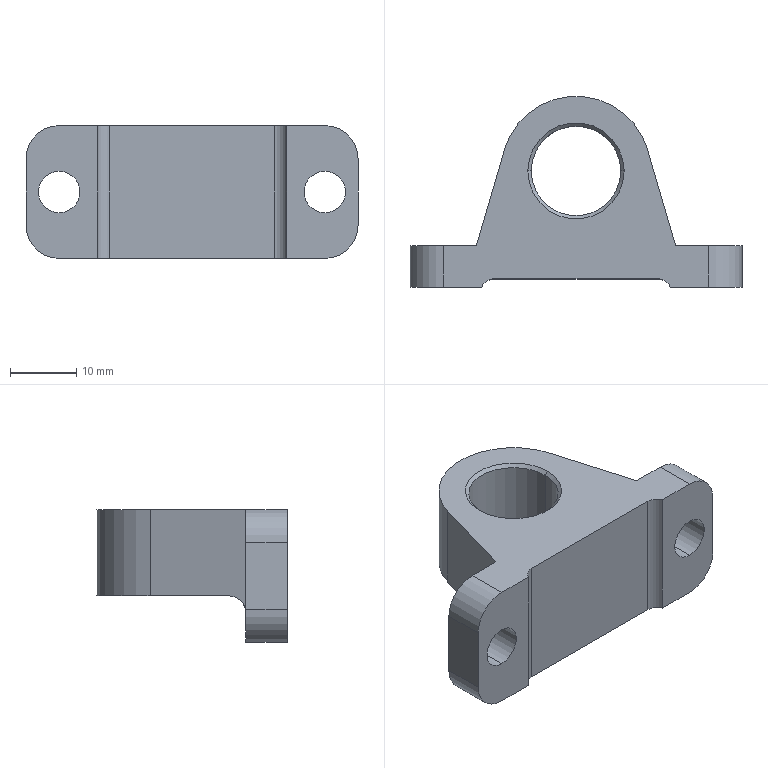Component | SolidWorks | CrankshaftSeat-1 | 1 solid | 29 faces | box 50 x 28.75 x 20 mm | volume 9719 mm3 | cylinder 14 | plane 11 | cone 4 | commonest cylinder face diameters 6.25 x4 10 x4 13.5 x2 4 x2 22.5 x1 5 x1
STEP:
#1=COLOUR_RGB('',0.7922,0.8196,0.9333);
#2=FILL_AREA_STYLE_COLOUR('',#1);
#3=FILL_AREA_STYLE('',(#2));
#4=SURFACE_STYLE_FILL_AREA(#3);
#5=SURFACE_SIDE_STYLE('',(#4));
#6=SURFACE_STYLE_USAGE(.BOTH.,#5);
#7=PRESENTATION_STYLE_ASSIGNMENT((#6));
#8=CARTESIAN_POINT('',(2.593,-9.906,9.939));
#9=VERTEX_POINT('',#8);
#10=CARTESIAN_POINT('',(3.125,-9.906,9.939));
#11=VERTEX_POINT('',#10);
#12=CARTESIAN_POINT('',(2.859,-9.906,9.939));
#13=DIRECTION('',(0.,0.,1.));
#14=DIRECTION('',(-1.,0.,0.));
#15=AXIS2_PLACEMENT_3D('',#12,#13,#14);
#16=CIRCLE('',#15,0.2657);
#17=EDGE_CURVE('',#9,#11,#16,.T.);
#18=ORIENTED_EDGE('',*,*,#17,.F.);
#19=CARTESIAN_POINT('',(2.573,-9.906,9.959));
#20=VERTEX_POINT('',#19);
#21=CARTESIAN_POINT('',(2.573,-9.906,9.959));
#22=DIRECTION('',(-0.7071,0.,0.7071));
#23=VECTOR('',#22,39.37);
#24=LINE('',#21,#23);
#25=EDGE_CURVE('',#9,#20,#24,.T.);
#26=ORIENTED_EDGE('',*,*,#25,.T.);
#27=CARTESIAN_POINT('',(3.144,-9.906,9.959));
#28=VERTEX_POINT('',#27);
#29=CARTESIAN_POINT('',(2.859,-9.906,9.959));
#30=DIRECTION('',(0.,0.,-1.));
#31=DIRECTION('',(-1.,0.,0.));
#32=AXIS2_PLACEMENT_3D('',#29,#30,#31);
#33=CIRCLE('',#32,0.2854);
#34=EDGE_CURVE('',#28,#20,#33,.T.);
#35=ORIENTED_EDGE('',*,*,#34,.F.);
#36=CARTESIAN_POINT('',(3.144,-9.906,9.959));
#37=DIRECTION('',(0.7071,0.,0.7071));
#38=VECTOR('',#37,39.37);
#39=LINE('',#36,#38);
#40=EDGE_CURVE('',#11,#28,#39,.T.);
#41=ORIENTED_EDGE('',*,*,#40,.F.);
#42=EDGE_LOOP('',(#18,#26,#35,#41));
#43=FACE_OUTER_BOUND('',#42,.T.);
#44=CARTESIAN_POINT('',(2.859,-9.906,9.959));
#45=DIRECTION('',(0.,0.,1.));
#46=DIRECTION('',(1.,0.,0.));
#47=AXIS2_PLACEMENT_3D('',#44,#45,#46);
#48=CONICAL_SURFACE('',#47,0.2854,0.7854);
#49=ADVANCED_FACE('',(#43),#48,.F.);
#50=CARTESIAN_POINT('',(3.125,-9.906,9.467));
#51=VERTEX_POINT('',#50);
#52=CARTESIAN_POINT('',(2.593,-9.906,9.467));
#53=VERTEX_POINT('',#52);
#54=CARTESIAN_POINT('',(2.859,-9.906,9.467));
#55=DIRECTION('',(0.,0.,-1.));
#56=DIRECTION('',(1.,0.,0.));
#57=AXIS2_PLACEMENT_3D('',#54,#55,#56);
#58=CIRCLE('',#57,0.2657);
#59=EDGE_CURVE('',#51,#53,#58,.T.);
#60=ORIENTED_EDGE('',*,*,#59,.F.);
#61=CARTESIAN_POINT('',(3.144,-9.906,9.447));
#62=VERTEX_POINT('',#61);
#63=CARTESIAN_POINT('',(3.144,-9.906,9.447));
#64=DIRECTION('',(0.7071,0.,-0.7071));
#65=VECTOR('',#64,39.37);
#66=LINE('',#63,#65);
#67=EDGE_CURVE('',#51,#62,#66,.T.);
#68=ORIENTED_EDGE('',*,*,#67,.T.);
#69=CARTESIAN_POINT('',(2.573,-9.906,9.447));
#70=VERTEX_POINT('',#69);
#71=CARTESIAN_POINT('',(2.859,-9.906,9.447));
#72=DIRECTION('',(0.,0.,1.));
#73=DIRECTION('',(1.,0.,0.));
#74=AXIS2_PLACEMENT_3D('',#71,#72,#73);
#75=CIRCLE('',#74,0.2854);
#76=EDGE_CURVE('',#70,#62,#75,.T.);
#77=ORIENTED_EDGE('',*,*,#76,.F.);
#78=CARTESIAN_POINT('',(2.573,-9.906,9.447));
#79=DIRECTION('',(-0.7071,0.,-0.7071));
#80=VECTOR('',#79,39.37);
#81=LINE('',#78,#80);
#82=EDGE_CURVE('',#53,#70,#81,.T.);
#83=ORIENTED_EDGE('',*,*,#82,.F.);
#84=EDGE_LOOP('',(#60,#68,#77,#83));
#85=FACE_OUTER_BOUND('',#84,.T.);
#86=CARTESIAN_POINT('',(2.859,-9.906,9.447));
#87=DIRECTION('',(0.,0.,-1.));
#88=DIRECTION('',(-1.,0.,0.));
#89=AXIS2_PLACEMENT_3D('',#86,#87,#88);
#90=CONICAL_SURFACE('',#89,0.2854,0.7854);
#91=ADVANCED_FACE('',(#85),#90,.F.);
#92=ORIENTED_EDGE('',*,*,#59,.T.);
#93=CARTESIAN_POINT('',(2.593,-9.906,9.447));
#94=DIRECTION('',(0.,0.,1.));
#95=VECTOR('',#94,39.37);
#96=LINE('',#93,#95);
#97=EDGE_CURVE('',#53,#9,#96,.T.);
#98=ORIENTED_EDGE('',*,*,#97,.T.);
#99=ORIENTED_EDGE('',*,*,#17,.T.);
#100=CARTESIAN_POINT('',(3.125,-9.906,9.447));
#101=DIRECTION('',(0.,0.,1.));
#102=VECTOR('',#101,39.37);
#103=LINE('',#100,#102);
#104=EDGE_CURVE('',#51,#11,#103,.T.);
#105=ORIENTED_EDGE('',*,*,#104,.F.);
#106=EDGE_LOOP('',(#92,#98,#99,#105));
#107=FACE_OUTER_BOUND('',#106,.T.);
#108=CARTESIAN_POINT('',(2.859,-9.906,9.447));
#109=DIRECTION('',(0.,0.,1.));
#110=DIRECTION('',(1.,0.,0.));
#111=AXIS2_PLACEMENT_3D('',#108,#109,#110);
#112=CYLINDRICAL_SURFACE('',#111,0.2657);
#113=ADVANCED_FACE('',(#107),#112,.F.);
#114=CARTESIAN_POINT('',(3.646,-10.594,9.442));
#115=VERTEX_POINT('',#114);
#116=CARTESIAN_POINT('',(3.646,-10.594,9.688));
#117=VERTEX_POINT('',#116);
#118=CARTESIAN_POINT('',(3.646,-10.594,9.565));
#119=DIRECTION('',(0.,1.,0.));
#120=DIRECTION('',(0.,0.,1.));
#121=AXIS2_PLACEMENT_3D('',#118,#119,#120);
#122=CIRCLE('',#121,0.123);
#123=EDGE_CURVE('',#115,#117,#122,.T.);
#124=ORIENTED_EDGE('',*,*,#123,.F.);
#125=CARTESIAN_POINT('',(3.646,-10.348,9.442));
#126=VERTEX_POINT('',#125);
#127=CARTESIAN_POINT('',(3.646,-10.594,9.442));
#128=DIRECTION('',(0.,1.,0.));
#129=VECTOR('',#128,39.37);
#130=LINE('',#127,#129);
#131=EDGE_CURVE('',#115,#126,#130,.T.);
#132=ORIENTED_EDGE('',*,*,#131,.T.);
#133=CARTESIAN_POINT('',(3.646,-10.348,9.688));
#134=VERTEX_POINT('',#133);
#135=CARTESIAN_POINT('',(3.646,-10.348,9.565));
#136=DIRECTION('',(0.,1.,0.));
#137=DIRECTION('',(0.,0.,1.));
#138=AXIS2_PLACEMENT_3D('',#135,#136,#137);
#139=CIRCLE('',#138,0.123);
#140=EDGE_CURVE('',#126,#134,#139,.T.);
#141=ORIENTED_EDGE('',*,*,#140,.T.);
#142=CARTESIAN_POINT('',(3.646,-10.594,9.688));
#143=DIRECTION('',(0.,1.,0.));
#144=VECTOR('',#143,39.37);
#145=LINE('',#142,#144);
#146=EDGE_CURVE('',#117,#134,#145,.T.);
#147=ORIENTED_EDGE('',*,*,#146,.F.);
#148=EDGE_LOOP('',(#124,#132,#141,#147));
#149=FACE_OUTER_BOUND('',#148,.T.);
#150=CARTESIAN_POINT('',(3.646,-10.594,9.565));
#151=DIRECTION('',(0.,1.,0.));
#152=DIRECTION('',(0.,0.,1.));
#153=AXIS2_PLACEMENT_3D('',#150,#151,#152);
#154=CYLINDRICAL_SURFACE('',#153,0.123);
#155=ADVANCED_FACE('',(#149),#154,.F.);
#156=CARTESIAN_POINT('',(2.072,-10.594,9.442));
#157=VERTEX_POINT('',#156);
#158=CARTESIAN_POINT('',(2.072,-10.594,9.688));
#159=VERTEX_POINT('',#158);
#160=CARTESIAN_POINT('',(2.072,-10.594,9.565));
#161=DIRECTION('',(0.,1.,0.));
#162=DIRECTION('',(0.,0.,1.));
#163=AXIS2_PLACEMENT_3D('',#160,#161,#162);
#164=CIRCLE('',#163,0.123);
#165=EDGE_CURVE('',#157,#159,#164,.T.);
#166=ORIENTED_EDGE('',*,*,#165,.F.);
#167=CARTESIAN_POINT('',(2.072,-10.348,9.442));
#168=VERTEX_POINT('',#167);
#169=CARTESIAN_POINT('',(2.072,-10.594,9.442));
#170=DIRECTION('',(0.,1.,0.));
#171=VECTOR('',#170,39.37);
#172=LINE('',#169,#171);
#173=EDGE_CURVE('',#157,#168,#172,.T.);
#174=ORIENTED_EDGE('',*,*,#173,.T.);
#175=CARTESIAN_POINT('',(2.072,-10.348,9.688));
#176=VERTEX_POINT('',#175);
#177=CARTESIAN_POINT('',(2.072,-10.348,9.565));
#178=DIRECTION('',(0.,1.,0.));
#179=DIRECTION('',(0.,0.,1.));
#180=AXIS2_PLACEMENT_3D('',#177,#178,#179);
#181=CIRCLE('',#180,0.123);
#182=EDGE_CURVE('',#168,#176,#181,.T.);
#183=ORIENTED_EDGE('',*,*,#182,.T.);
#184=CARTESIAN_POINT('',(2.072,-10.594,9.688));
#185=DIRECTION('',(0.,1.,0.));
#186=VECTOR('',#185,39.37);
#187=LINE('',#184,#186);
#188=EDGE_CURVE('',#159,#176,#187,.T.);
#189=ORIENTED_EDGE('',*,*,#188,.F.);
#190=EDGE_LOOP('',(#166,#174,#183,#189));
#191=FACE_OUTER_BOUND('',#190,.T.);
#192=CARTESIAN_POINT('',(2.072,-10.594,9.565));
#193=DIRECTION('',(0.,1.,0.));
#194=DIRECTION('',(0.,0.,1.));
#195=AXIS2_PLACEMENT_3D('',#192,#193,#194);
#196=CYLINDRICAL_SURFACE('',#195,0.123);
#197=ADVANCED_FACE('',(#191),#196,.F.);
#198=CARTESIAN_POINT('',(3.42,-10.594,9.172));
#199=VERTEX_POINT('',#198);
#200=CARTESIAN_POINT('',(3.42,-10.594,9.959));
#201=VERTEX_POINT('',#200);
#202=CARTESIAN_POINT('',(3.42,-10.594,9.565));
#203=DIRECTION('',(0.,0.,1.));
#204=VECTOR('',#203,39.37);
#205=LINE('',#202,#204);
#206=EDGE_CURVE('',#199,#201,#205,.T.);
#207=ORIENTED_EDGE('',*,*,#206,.F.);
#208=CARTESIAN_POINT('',(3.646,-10.594,9.172));
#209=VERTEX_POINT('',#208);
#210=CARTESIAN_POINT('',(1.875,-10.594,9.172));
#211=DIRECTION('',(-1.,0.,0.));
#212=VECTOR('',#211,39.37);
#213=LINE('',#210,#212);
#214=EDGE_CURVE('',#209,#199,#213,.T.);
#215=ORIENTED_EDGE('',*,*,#214,.F.);
#216=CARTESIAN_POINT('',(3.843,-10.594,9.369));
#217=VERTEX_POINT('',#216);
#218=CARTESIAN_POINT('',(3.646,-10.594,9.369));
#219=DIRECTION('',(0.,-1.,0.));
#220=DIRECTION('',(0.,0.,-1.));
#221=AXIS2_PLACEMENT_3D('',#218,#219,#220);
#222=CIRCLE('',#221,0.1969);
#223=EDGE_CURVE('',#209,#217,#222,.T.);
#224=ORIENTED_EDGE('',*,*,#223,.T.);
#225=CARTESIAN_POINT('',(3.843,-10.594,9.762));
#226=VERTEX_POINT('',#225);
#227=CARTESIAN_POINT('',(3.843,-10.594,9.959));
#228=DIRECTION('',(0.,0.,-1.));
#229=VECTOR('',#228,39.37);
#230=LINE('',#227,#229);
#231=EDGE_CURVE('',#226,#217,#230,.T.);
#232=ORIENTED_EDGE('',*,*,#231,.F.);
#233=CARTESIAN_POINT('',(3.646,-10.594,9.959));
#234=VERTEX_POINT('',#233);
#235=CARTESIAN_POINT('',(3.646,-10.594,9.762));
#236=DIRECTION('',(0.,-1.,0.));
#237=DIRECTION('',(0.,0.,-1.));
#238=AXIS2_PLACEMENT_3D('',#235,#236,#237);
#239=CIRCLE('',#238,0.1969);
#240=EDGE_CURVE('',#226,#234,#239,.T.);
#241=ORIENTED_EDGE('',*,*,#240,.T.);
#242=CARTESIAN_POINT('',(1.875,-10.594,9.959));
#243=DIRECTION('',(1.,0.,0.));
#244=VECTOR('',#243,39.37);
#245=LINE('',#242,#244);
#246=EDGE_CURVE('',#201,#234,#245,.T.);
#247=ORIENTED_EDGE('',*,*,#246,.F.);
#248=EDGE_LOOP('',(#207,#215,#224,#232,#241,#247));
#249=FACE_OUTER_BOUND('',#248,.T.);
#250=CARTESIAN_POINT('',(3.646,-10.594,9.565));
#251=DIRECTION('',(0.,1.,0.));
#252=DIRECTION('',(0.,0.,1.));
#253=AXIS2_PLACEMENT_3D('',#250,#251,#252);
#254=CIRCLE('',#253,0.123);
#255=EDGE_CURVE('',#117,#115,#254,.T.);
#256=ORIENTED_EDGE('',*,*,#255,.T.);
#257=ORIENTED_EDGE('',*,*,#123,.T.);
#258=EDGE_LOOP('',(#256,#257));
#259=FACE_BOUND('',#258,.T.);
#260=CARTESIAN_POINT('',(2.859,-10.594,9.565));
#261=DIRECTION('',(0.,-1.,0.));
#262=DIRECTION('',(0.,0.,-1.));
#263=AXIS2_PLACEMENT_3D('',#260,#261,#262);
#264=PLANE('',#263);
#265=ADVANCED_FACE('',(#249,#259),#264,.T.);
#266=CARTESIAN_POINT('',(3.843,-10.348,9.762));
#267=VERTEX_POINT('',#266);
#268=CARTESIAN_POINT('',(3.843,-10.348,9.369));
#269=VERTEX_POINT('',#268);
#270=CARTESIAN_POINT('',(3.843,-10.348,9.959));
#271=DIRECTION('',(0.,0.,-1.));
#272=VECTOR('',#271,39.37);
#273=LINE('',#270,#272);
#274=EDGE_CURVE('',#267,#269,#273,.T.);
#275=ORIENTED_EDGE('',*,*,#274,.F.);
#276=CARTESIAN_POINT('',(3.843,-10.348,9.762));
#277=DIRECTION('',(0.,-1.,0.));
#278=VECTOR('',#277,39.37);
#279=LINE('',#276,#278);
#280=EDGE_CURVE('',#267,#226,#279,.T.);
#281=ORIENTED_EDGE('',*,*,#280,.T.);
#282=ORIENTED_EDGE('',*,*,#231,.T.);
#283=CARTESIAN_POINT('',(3.843,-10.348,9.369));
#284=DIRECTION('',(0.,1.,0.));
#285=VECTOR('',#284,39.37);
#286=LINE('',#283,#285);
#287=EDGE_CURVE('',#217,#269,#286,.T.);
#288=ORIENTED_EDGE('',*,*,#287,.T.);
#289=EDGE_LOOP('',(#275,#281,#282,#288));
#290=FACE_OUTER_BOUND('',#289,.T.);
#291=CARTESIAN_POINT('',(3.843,-10.348,9.959));
#292=DIRECTION('',(-1.,0.,0.));
#293=DIRECTION('',(0.,0.,1.));
#294=AXIS2_PLACEMENT_3D('',#291,#292,#293);
#295=PLANE('',#294);
#296=ADVANCED_FACE('',(#290),#295,.F.);
#297=ORIENTED_EDGE('',*,*,#214,.T.);
#298=CARTESIAN_POINT('',(3.347,-10.545,9.172));
#299=VERTEX_POINT('',#298);
#300=CARTESIAN_POINT('',(3.347,-10.624,9.172));
#301=DIRECTION('',(0.,0.,1.));
#302=DIRECTION('',(1.,0.,0.));
#303=AXIS2_PLACEMENT_3D('',#300,#301,#302);
#304=CIRCLE('',#303,0.07874);
#305=EDGE_CURVE('',#199,#299,#304,.T.);
#306=ORIENTED_EDGE('',*,*,#305,.T.);
#307=CARTESIAN_POINT('',(2.371,-10.545,9.172));
#308=VERTEX_POINT('',#307);
#309=CARTESIAN_POINT('',(2.298,-10.545,9.172));
#310=DIRECTION('',(-1.,0.,0.));
#311=VECTOR('',#310,39.37);
#312=LINE('',#309,#311);
#313=EDGE_CURVE('',#299,#308,#312,.T.);
#314=ORIENTED_EDGE('',*,*,#313,.T.);
#315=CARTESIAN_POINT('',(2.298,-10.594,9.172));
#316=VERTEX_POINT('',#315);
#317=CARTESIAN_POINT('',(2.371,-10.624,9.172));
#318=DIRECTION('',(0.,0.,1.));
#319=DIRECTION('',(1.,0.,0.));
#320=AXIS2_PLACEMENT_3D('',#317,#318,#319);
#321=CIRCLE('',#320,0.07874);
#322=EDGE_CURVE('',#308,#316,#321,.T.);
#323=ORIENTED_EDGE('',*,*,#322,.T.);
#324=CARTESIAN_POINT('',(2.072,-10.594,9.172));
#325=VERTEX_POINT('',#324);
#326=CARTESIAN_POINT('',(1.875,-10.594,9.172));
#327=DIRECTION('',(-1.,0.,0.));
#328=VECTOR('',#327,39.37);
#329=LINE('',#326,#328);
#330=EDGE_CURVE('',#316,#325,#329,.T.);
#331=ORIENTED_EDGE('',*,*,#330,.T.);
#332=CARTESIAN_POINT('',(2.072,-10.348,9.172));
#333=VERTEX_POINT('',#332);
#334=CARTESIAN_POINT('',(2.072,-10.348,9.172));
#335=DIRECTION('',(0.,1.,0.));
#336=VECTOR('',#335,39.37);
#337=LINE('',#334,#336);
#338=EDGE_CURVE('',#325,#333,#337,.T.);
#339=ORIENTED_EDGE('',*,*,#338,.T.);
#340=CARTESIAN_POINT('',(3.646,-10.348,9.172));
#341=VERTEX_POINT('',#340);
#342=CARTESIAN_POINT('',(1.875,-10.348,9.172));
#343=DIRECTION('',(-1.,0.,0.));
#344=VECTOR('',#343,39.37);
#345=LINE('',#342,#344);
#346=EDGE_CURVE('',#341,#333,#345,.T.);
#347=ORIENTED_EDGE('',*,*,#346,.F.);
#348=CARTESIAN_POINT('',(3.646,-10.348,9.172));
#349=DIRECTION('',(0.,-1.,0.));
#350=VECTOR('',#349,39.37);
#351=LINE('',#348,#350);
#352=EDGE_CURVE('',#341,#209,#351,.T.);
#353=ORIENTED_EDGE('',*,*,#352,.T.);
#354=EDGE_LOOP('',(#297,#306,#314,#323,#331,#339,#347,#353));
#355=FACE_OUTER_BOUND('',#354,.T.);
#356=CARTESIAN_POINT('',(1.875,-10.348,9.172));
#357=DIRECTION('',(0.,0.,1.));
#358=DIRECTION('',(1.,0.,0.));
#359=AXIS2_PLACEMENT_3D('',#356,#357,#358);
#360=PLANE('',#359);
#361=ADVANCED_FACE('',(#355),#360,.F.);
#362=CARTESIAN_POINT('',(1.875,-10.594,9.369));
#363=VERTEX_POINT('',#362);
#364=CARTESIAN_POINT('',(1.875,-10.594,9.762));
#365=VERTEX_POINT('',#364);
#366=CARTESIAN_POINT('',(1.875,-10.594,9.959));
#367=DIRECTION('',(0.,0.,1.));
#368=VECTOR('',#367,39.37);
#369=LINE('',#366,#368);
#370=EDGE_CURVE('',#363,#365,#369,.T.);
#371=ORIENTED_EDGE('',*,*,#370,.T.);
#372=CARTESIAN_POINT('',(1.875,-10.348,9.762));
#373=VERTEX_POINT('',#372);
#374=CARTESIAN_POINT('',(1.875,-10.348,9.762));
#375=DIRECTION('',(0.,1.,0.));
#376=VECTOR('',#375,39.37);
#377=LINE('',#374,#376);
#378=EDGE_CURVE('',#365,#373,#377,.T.);
#379=ORIENTED_EDGE('',*,*,#378,.T.);
#380=CARTESIAN_POINT('',(1.875,-10.348,9.369));
#381=VERTEX_POINT('',#380);
#382=CARTESIAN_POINT('',(1.875,-10.348,9.959));
#383=DIRECTION('',(0.,0.,1.));
#384=VECTOR('',#383,39.37);
#385=LINE('',#382,#384);
#386=EDGE_CURVE('',#381,#373,#385,.T.);
#387=ORIENTED_EDGE('',*,*,#386,.F.);
#388=CARTESIAN_POINT('',(1.875,-10.348,9.369));
#389=DIRECTION('',(0.,-1.,0.));
#390=VECTOR('',#389,39.37);
#391=LINE('',#388,#390);
#392=EDGE_CURVE('',#381,#363,#391,.T.);
#393=ORIENTED_EDGE('',*,*,#392,.T.);
#394=EDGE_LOOP('',(#371,#379,#387,#393));
#395=FACE_OUTER_BOUND('',#394,.T.);
#396=CARTESIAN_POINT('',(1.875,-10.348,9.959));
#397=DIRECTION('',(1.,0.,0.));
#398=DIRECTION('',(0.,0.,-1.));
#399=AXIS2_PLACEMENT_3D('',#396,#397,#398);
#400=PLANE('',#399);
#401=ADVANCED_FACE('',(#395),#400,.F.);
#402=ORIENTED_EDGE('',*,*,#34,.T.);
#403=CARTESIAN_POINT('',(2.859,-9.906,9.959));
#404=DIRECTION('',(0.,0.,-1.));
#405=DIRECTION('',(-1.,0.,0.));
#406=AXIS2_PLACEMENT_3D('',#403,#404,#405);
#407=CIRCLE('',#406,0.2854);
#408=EDGE_CURVE('',#20,#28,#407,.T.);
#409=ORIENTED_EDGE('',*,*,#408,.T.);
#410=EDGE_LOOP('',(#402,#409));
#411=FACE_BOUND('',#410,.T.);
#412=CARTESIAN_POINT('',(3.347,-10.545,9.959));
#413=VERTEX_POINT('',#412);
#414=CARTESIAN_POINT('',(2.371,-10.545,9.959));
#415=VERTEX_POINT('',#414);
#416=CARTESIAN_POINT('',(2.298,-10.545,9.959));
#417=DIRECTION('',(-1.,0.,0.));
#418=VECTOR('',#417,39.37);
#419=LINE('',#416,#418);
#420=EDGE_CURVE('',#413,#415,#419,.T.);
#421=ORIENTED_EDGE('',*,*,#420,.F.);
#422=CARTESIAN_POINT('',(3.347,-10.624,9.959));
#423=DIRECTION('',(0.,0.,-1.));
#424=DIRECTION('',(-1.,0.,0.));
#425=AXIS2_PLACEMENT_3D('',#422,#423,#424);
#426=CIRCLE('',#425,0.07874);
#427=EDGE_CURVE('',#413,#201,#426,.T.);
#428=ORIENTED_EDGE('',*,*,#427,.T.);
#429=ORIENTED_EDGE('',*,*,#246,.T.);
#430=CARTESIAN_POINT('',(3.646,-10.348,9.959));
#431=VERTEX_POINT('',#430);
#432=CARTESIAN_POINT('',(3.646,-10.348,9.959));
#433=DIRECTION('',(0.,1.,0.));
#434=VECTOR('',#433,39.37);
#435=LINE('',#432,#434);
#436=EDGE_CURVE('',#234,#431,#435,.T.);
#437=ORIENTED_EDGE('',*,*,#436,.T.);
#438=CARTESIAN_POINT('',(3.449,-10.348,9.959));
#439=VERTEX_POINT('',#438);
#440=CARTESIAN_POINT('',(1.875,-10.348,9.959));
#441=DIRECTION('',(1.,0.,0.));
#442=VECTOR('',#441,39.37);
#443=LINE('',#440,#442);
#444=EDGE_CURVE('',#439,#431,#443,.T.);
#445=ORIENTED_EDGE('',*,*,#444,.F.);
#446=CARTESIAN_POINT('',(3.284,-9.781,9.959));
#447=VERTEX_POINT('',#446);
#448=CARTESIAN_POINT('',(3.449,-10.348,9.959));
#449=DIRECTION('',(0.28,-0.96,0.));
#450=VECTOR('',#449,39.37);
#451=LINE('',#448,#450);
#452=EDGE_CURVE('',#447,#439,#451,.T.);
#453=ORIENTED_EDGE('',*,*,#452,.F.);
#454=CARTESIAN_POINT('',(2.434,-9.781,9.959));
#455=VERTEX_POINT('',#454);
#456=CARTESIAN_POINT('',(2.859,-9.906,9.959));
#457=DIRECTION('',(0.,0.,-1.));
#458=DIRECTION('',(-1.,0.,0.));
#459=AXIS2_PLACEMENT_3D('',#456,#457,#458);
#460=CIRCLE('',#459,0.4429);
#461=EDGE_CURVE('',#455,#447,#460,.T.);
#462=ORIENTED_EDGE('',*,*,#461,.F.);
#463=CARTESIAN_POINT('',(2.268,-10.348,9.959));
#464=VERTEX_POINT('',#463);
#465=CARTESIAN_POINT('',(2.268,-10.348,9.959));
#466=DIRECTION('',(0.28,0.96,0.));
#467=VECTOR('',#466,39.37);
#468=LINE('',#465,#467);
#469=EDGE_CURVE('',#464,#455,#468,.T.);
#470=ORIENTED_EDGE('',*,*,#469,.F.);
#471=CARTESIAN_POINT('',(2.072,-10.348,9.959));
#472=VERTEX_POINT('',#471);
#473=CARTESIAN_POINT('',(1.875,-10.348,9.959));
#474=DIRECTION('',(1.,0.,0.));
#475=VECTOR('',#474,39.37);
#476=LINE('',#473,#475);
#477=EDGE_CURVE('',#472,#464,#476,.T.);
#478=ORIENTED_EDGE('',*,*,#477,.F.);
#479=CARTESIAN_POINT('',(2.072,-10.594,9.959));
#480=VERTEX_POINT('',#479);
#481=CARTESIAN_POINT('',(2.072,-10.348,9.959));
#482=DIRECTION('',(0.,-1.,0.));
#483=VECTOR('',#482,39.37);
#484=LINE('',#481,#483);
#485=EDGE_CURVE('',#472,#480,#484,.T.);
#486=ORIENTED_EDGE('',*,*,#485,.T.);
#487=CARTESIAN_POINT('',(2.298,-10.594,9.959));
#488=VERTEX_POINT('',#487);
#489=CARTESIAN_POINT('',(1.875,-10.594,9.959));
#490=DIRECTION('',(1.,0.,0.));
#491=VECTOR('',#490,39.37);
#492=LINE('',#489,#491);
#493=EDGE_CURVE('',#480,#488,#492,.T.);
#494=ORIENTED_EDGE('',*,*,#493,.T.);
#495=CARTESIAN_POINT('',(2.371,-10.624,9.959));
#496=DIRECTION('',(0.,0.,-1.));
#497=DIRECTION('',(-1.,0.,0.));
#498=AXIS2_PLACEMENT_3D('',#495,#496,#497);
#499=CIRCLE('',#498,0.07874);
#500=EDGE_CURVE('',#488,#415,#499,.T.);
#501=ORIENTED_EDGE('',*,*,#500,.T.);
#502=EDGE_LOOP('',(#421,#428,#429,#437,#445,#453,#462,#470,#478,#486,#494,#501));
#503=FACE_OUTER_BOUND('',#502,.T.);
#504=CARTESIAN_POINT('',(1.875,-10.348,9.959));
#505=DIRECTION('',(0.,0.,-1.));
#506=DIRECTION('',(-1.,0.,0.));
#507=AXIS2_PLACEMENT_3D('',#504,#505,#506);
#508=PLANE('',#507);
#509=ADVANCED_FACE('',(#411,#503),#508,.F.);
#510=CARTESIAN_POINT('',(2.268,-10.348,9.349));
#511=VERTEX_POINT('',#510);
#512=CARTESIAN_POINT('',(3.449,-10.348,9.349));
#513=VERTEX_POINT('',#512);
#514=CARTESIAN_POINT('',(3.449,-10.348,9.349));
#515=DIRECTION('',(1.,0.,0.));
#516=VECTOR('',#515,39.37);
#517=LINE('',#514,#516);
#518=EDGE_CURVE('',#511,#513,#517,.T.);
#519=ORIENTED_EDGE('',*,*,#518,.T.);
#520=CARTESIAN_POINT('',(3.449,-10.348,9.447));
#521=DIRECTION('',(0.,0.,1.));
#522=VECTOR('',#521,39.37);
#523=LINE('',#520,#522);
#524=EDGE_CURVE('',#513,#439,#523,.T.);
#525=ORIENTED_EDGE('',*,*,#524,.T.);
#526=ORIENTED_EDGE('',*,*,#444,.T.);
#527=CARTESIAN_POINT('',(3.646,-10.348,9.762));
#528=DIRECTION('',(0.,1.,0.));
#529=DIRECTION('',(0.,0.,-1.));
#530=AXIS2_PLACEMENT_3D('',#527,#528,#529);
#531=CIRCLE('',#530,0.1969);
#532=EDGE_CURVE('',#431,#267,#531,.T.);
#533=ORIENTED_EDGE('',*,*,#532,.T.);
#534=ORIENTED_EDGE('',*,*,#274,.T.);
#535=CARTESIAN_POINT('',(3.646,-10.348,9.369));
#536=DIRECTION('',(0.,1.,0.));
#537=DIRECTION('',(0.,0.,-1.));
#538=AXIS2_PLACEMENT_3D('',#535,#536,#537);
#539=CIRCLE('',#538,0.1969);
#540=EDGE_CURVE('',#269,#341,#539,.T.);
#541=ORIENTED_EDGE('',*,*,#540,.T.);
#542=ORIENTED_EDGE('',*,*,#346,.T.);
#543=CARTESIAN_POINT('',(2.072,-10.348,9.369));
#544=DIRECTION('',(0.,1.,0.));
#545=DIRECTION('',(0.,0.,-1.));
#546=AXIS2_PLACEMENT_3D('',#543,#544,#545);
#547=CIRCLE('',#546,0.1969);
#548=EDGE_CURVE('',#333,#381,#547,.T.);
#549=ORIENTED_EDGE('',*,*,#548,.T.);
#550=ORIENTED_EDGE('',*,*,#386,.T.);
#551=CARTESIAN_POINT('',(2.072,-10.348,9.762));
#552=DIRECTION('',(0.,1.,0.));
#553=DIRECTION('',(0.,0.,-1.));
#554=AXIS2_PLACEMENT_3D('',#551,#552,#553);
#555=CIRCLE('',#554,0.1969);
#556=EDGE_CURVE('',#373,#472,#555,.T.);
#557=ORIENTED_EDGE('',*,*,#556,.T.);
#558=ORIENTED_EDGE('',*,*,#477,.T.);
#559=CARTESIAN_POINT('',(2.268,-10.348,9.447));
#560=DIRECTION('',(0.,0.,1.));
#561=VECTOR('',#560,39.37);
#562=LINE('',#559,#561);
#563=EDGE_CURVE('',#511,#464,#562,.T.);
#564=ORIENTED_EDGE('',*,*,#563,.F.);
#565=EDGE_LOOP('',(#519,#525,#526,#533,#534,#541,#542,#549,#550,#557,#558,#564));
#566=FACE_OUTER_BOUND('',#565,.T.);
#567=CARTESIAN_POINT('',(3.646,-10.348,9.565));
#568=DIRECTION('',(0.,1.,0.));
#569=DIRECTION('',(0.,0.,1.));
#570=AXIS2_PLACEMENT_3D('',#567,#568,#569);
#571=CIRCLE('',#570,0.123);
#572=EDGE_CURVE('',#134,#126,#571,.T.);
#573=ORIENTED_EDGE('',*,*,#572,.F.);
#574=ORIENTED_EDGE('',*,*,#140,.F.);
#575=EDGE_LOOP('',(#573,#574));
#576=FACE_BOUND('',#575,.T.);
#577=CARTESIAN_POINT('',(2.072,-10.348,9.565));
#578=DIRECTION('',(0.,1.,0.));
#579=DIRECTION('',(0.,0.,1.));
#580=AXIS2_PLACEMENT_3D('',#577,#578,#579);
#581=CIRCLE('',#580,0.123);
#582=EDGE_CURVE('',#176,#168,#581,.T.);
#583=ORIENTED_EDGE('',*,*,#582,.F.);
#584=ORIENTED_EDGE('',*,*,#182,.F.);
#585=EDGE_LOOP('',(#583,#584));
#586=FACE_BOUND('',#585,.T.);
#587=CARTESIAN_POINT('',(2.859,-10.348,9.565));
#588=DIRECTION('',(0.,-1.,0.));
#589=DIRECTION('',(0.,0.,-1.));
#590=AXIS2_PLACEMENT_3D('',#587,#588,#589);
#591=PLANE('',#590);
#592=ADVANCED_FACE('',(#566,#576,#586),#591,.F.);
#593=CARTESIAN_POINT('',(2.298,-10.594,9.565));
#594=DIRECTION('',(0.,0.,-1.));
#595=VECTOR('',#594,39.37);
#596=LINE('',#593,#595);
#597=EDGE_CURVE('',#488,#316,#596,.T.);
#598=ORIENTED_EDGE('',*,*,#597,.F.);
#599=ORIENTED_EDGE('',*,*,#493,.F.);
#600=CARTESIAN_POINT('',(2.072,-10.594,9.762));
#601=DIRECTION('',(0.,-1.,0.));
#602=DIRECTION('',(0.,0.,-1.));
#603=AXIS2_PLACEMENT_3D('',#600,#601,#602);
#604=CIRCLE('',#603,0.1969);
#605=EDGE_CURVE('',#480,#365,#604,.T.);
#606=ORIENTED_EDGE('',*,*,#605,.T.);
#607=ORIENTED_EDGE('',*,*,#370,.F.);
#608=CARTESIAN_POINT('',(2.072,-10.594,9.369));
#609=DIRECTION('',(0.,-1.,0.));
#610=DIRECTION('',(0.,0.,-1.));
#611=AXIS2_PLACEMENT_3D('',#608,#609,#610);
#612=CIRCLE('',#611,0.1969);
#613=EDGE_CURVE('',#363,#325,#612,.T.);
#614=ORIENTED_EDGE('',*,*,#613,.T.);
#615=ORIENTED_EDGE('',*,*,#330,.F.);
#616=EDGE_LOOP('',(#598,#599,#606,#607,#614,#615));
#617=FACE_OUTER_BOUND('',#616,.T.);
#618=CARTESIAN_POINT('',(2.072,-10.594,9.565));
#619=DIRECTION('',(0.,1.,0.));
#620=DIRECTION('',(0.,0.,1.));
#621=AXIS2_PLACEMENT_3D('',#618,#619,#620);
#622=CIRCLE('',#621,0.123);
#623=EDGE_CURVE('',#159,#157,#622,.T.);
#624=ORIENTED_EDGE('',*,*,#623,.T.);
#625=ORIENTED_EDGE('',*,*,#165,.T.);
#626=EDGE_LOOP('',(#624,#625));
#627=FACE_BOUND('',#626,.T.);
#628=CARTESIAN_POINT('',(2.859,-10.594,9.565));
#629=DIRECTION('',(0.,-1.,0.));
#630=DIRECTION('',(0.,0.,-1.));
#631=AXIS2_PLACEMENT_3D('',#628,#629,#630);
#632=PLANE('',#631);
#633=ADVANCED_FACE('',(#617,#627),#632,.T.);
#634=ORIENTED_EDGE('',*,*,#173,.F.);
#635=ORIENTED_EDGE('',*,*,#623,.F.);
#636=ORIENTED_EDGE('',*,*,#188,.T.);
#637=ORIENTED_EDGE('',*,*,#582,.T.);
#638=EDGE_LOOP('',(#634,#635,#636,#637));
#639=FACE_OUTER_BOUND('',#638,.T.);
#640=CARTESIAN_POINT('',(2.072,-10.594,9.565));
#641=DIRECTION('',(0.,1.,0.));
#642=DIRECTION('',(0.,0.,1.));
#643=AXIS2_PLACEMENT_3D('',#640,#641,#642);
#644=CYLINDRICAL_SURFACE('',#643,0.123);
#645=ADVANCED_FACE('',(#639),#644,.F.);
#646=ORIENTED_EDGE('',*,*,#131,.F.);
#647=ORIENTED_EDGE('',*,*,#255,.F.);
#648=ORIENTED_EDGE('',*,*,#146,.T.);
#649=ORIENTED_EDGE('',*,*,#572,.T.);
#650=EDGE_LOOP('',(#646,#647,#648,#649));
#651=FACE_OUTER_BOUND('',#650,.T.);
#652=CARTESIAN_POINT('',(3.646,-10.594,9.565));
#653=DIRECTION('',(0.,1.,0.));
#654=DIRECTION('',(0.,0.,1.));
#655=AXIS2_PLACEMENT_3D('',#652,#653,#654);
#656=CYLINDRICAL_SURFACE('',#655,0.123);
#657=ADVANCED_FACE('',(#651),#656,.F.);
#658=ORIENTED_EDGE('',*,*,#563,.T.);
#659=ORIENTED_EDGE('',*,*,#469,.T.);
#660=CARTESIAN_POINT('',(2.434,-9.781,9.447));
#661=VERTEX_POINT('',#660);
#662=CARTESIAN_POINT('',(2.434,-9.781,9.447));
#663=DIRECTION('',(0.,0.,1.));
#664=VECTOR('',#663,39.37);
#665=LINE('',#662,#664);
#666=EDGE_CURVE('',#661,#455,#665,.T.);
#667=ORIENTED_EDGE('',*,*,#666,.F.);
#668=CARTESIAN_POINT('',(2.297,-10.25,9.447));
#669=VERTEX_POINT('',#668);
#670=CARTESIAN_POINT('',(2.268,-10.348,9.447));
#671=DIRECTION('',(-0.28,-0.96,0.));
#672=VECTOR('',#671,39.37);
#673=LINE('',#670,#672);
#674=EDGE_CURVE('',#661,#669,#673,.T.);
#675=ORIENTED_EDGE('',*,*,#674,.T.);
#676=CARTESIAN_POINT('',(2.297,-10.25,9.447));
#677=CARTESIAN_POINT('',(2.28,-10.308,9.447));
#678=CARTESIAN_POINT('',(2.268,-10.348,9.407));
#679=CARTESIAN_POINT('',(2.268,-10.348,9.349));
#680=(BOUNDED_CURVE()B_SPLINE_CURVE(3,(#676,#677,#678,#679),.UNSPECIFIED.,.F.,.F.)B_SPLINE_CURVE_WITH_KNOTS((4,4),(4.712,6.283),.UNSPECIFIED.)CURVE()GEOMETRIC_REPRESENTATION_ITEM()RATIONAL_B_SPLINE_CURVE((1.,0.8047,0.8047,1.))REPRESENTATION_ITEM(''));
#681=EDGE_CURVE('',#669,#511,#680,.T.);
#682=ORIENTED_EDGE('',*,*,#681,.T.);
#683=EDGE_LOOP('',(#658,#659,#667,#675,#682));
#684=FACE_OUTER_BOUND('',#683,.T.);
#685=CARTESIAN_POINT('',(2.268,-10.348,9.447));
#686=DIRECTION('',(-0.96,0.28,0.));
#687=DIRECTION('',(-0.28,-0.96,0.));
#688=AXIS2_PLACEMENT_3D('',#685,#686,#687);
#689=PLANE('',#688);
#690=ADVANCED_FACE('',(#684),#689,.T.);
#691=ORIENTED_EDGE('',*,*,#666,.T.);
#692=ORIENTED_EDGE('',*,*,#461,.T.);
#693=CARTESIAN_POINT('',(3.284,-9.781,9.447));
#694=VERTEX_POINT('',#693);
#695=CARTESIAN_POINT('',(3.284,-9.781,9.447));
#696=DIRECTION('',(0.,0.,1.));
#697=VECTOR('',#696,39.37);
#698=LINE('',#695,#697);
#699=EDGE_CURVE('',#694,#447,#698,.T.);
#700=ORIENTED_EDGE('',*,*,#699,.F.);
#701=CARTESIAN_POINT('',(2.859,-9.906,9.447));
#702=DIRECTION('',(0.,0.,1.));
#703=DIRECTION('',(1.,0.,0.));
#704=AXIS2_PLACEMENT_3D('',#701,#702,#703);
#705=CIRCLE('',#704,0.4429);
#706=EDGE_CURVE('',#694,#661,#705,.T.);
#707=ORIENTED_EDGE('',*,*,#706,.T.);
#708=EDGE_LOOP('',(#691,#692,#700,#707));
#709=FACE_OUTER_BOUND('',#708,.T.);
#710=CARTESIAN_POINT('',(2.859,-9.906,9.447));
#711=DIRECTION('',(0.,0.,1.));
#712=DIRECTION('',(1.,0.,0.));
#713=AXIS2_PLACEMENT_3D('',#710,#711,#712);
#714=CYLINDRICAL_SURFACE('',#713,0.4429);
#715=ADVANCED_FACE('',(#709),#714,.T.);
#716=ORIENTED_EDGE('',*,*,#699,.T.);
#717=ORIENTED_EDGE('',*,*,#452,.T.);
#718=ORIENTED_EDGE('',*,*,#524,.F.);
#719=CARTESIAN_POINT('',(3.421,-10.25,9.447));
#720=VERTEX_POINT('',#719);
#721=CARTESIAN_POINT('',(3.449,-10.348,9.349));
#722=CARTESIAN_POINT('',(3.449,-10.348,9.407));
#723=CARTESIAN_POINT('',(3.438,-10.308,9.447));
#724=CARTESIAN_POINT('',(3.421,-10.25,9.447));
#725=(BOUNDED_CURVE()B_SPLINE_CURVE(3,(#721,#722,#723,#724),.UNSPECIFIED.,.F.,.F.)B_SPLINE_CURVE_WITH_KNOTS((4,4),(3.142,4.712),.UNSPECIFIED.)CURVE()GEOMETRIC_REPRESENTATION_ITEM()RATIONAL_B_SPLINE_CURVE((1.,0.8047,0.8047,1.))REPRESENTATION_ITEM(''));
#726=EDGE_CURVE('',#513,#720,#725,.T.);
#727=ORIENTED_EDGE('',*,*,#726,.T.);
#728=CARTESIAN_POINT('',(3.449,-10.348,9.447));
#729=DIRECTION('',(-0.28,0.96,0.));
#730=VECTOR('',#729,39.37);
#731=LINE('',#728,#730);
#732=EDGE_CURVE('',#720,#694,#731,.T.);
#733=ORIENTED_EDGE('',*,*,#732,.T.);
#734=EDGE_LOOP('',(#716,#717,#718,#727,#733));
#735=FACE_OUTER_BOUND('',#734,.T.);
#736=CARTESIAN_POINT('',(3.449,-10.348,9.447));
#737=DIRECTION('',(0.96,0.28,0.));
#738=DIRECTION('',(-0.28,0.96,0.));
#739=AXIS2_PLACEMENT_3D('',#736,#737,#738);
#740=PLANE('',#739);
#741=ADVANCED_FACE('',(#735),#740,.T.);
#742=ORIENTED_EDGE('',*,*,#76,.T.);
#743=CARTESIAN_POINT('',(2.859,-9.906,9.447));
#744=DIRECTION('',(0.,0.,1.));
#745=DIRECTION('',(1.,0.,0.));
#746=AXIS2_PLACEMENT_3D('',#743,#744,#745);
#747=CIRCLE('',#746,0.2854);
#748=EDGE_CURVE('',#62,#70,#747,.T.);
#749=ORIENTED_EDGE('',*,*,#748,.T.);
#750=EDGE_LOOP('',(#742,#749));
#751=FACE_BOUND('',#750,.T.);
#752=ORIENTED_EDGE('',*,*,#732,.F.);
#753=CARTESIAN_POINT('',(2.268,-10.25,9.447));
#754=DIRECTION('',(-1.,0.,0.));
#755=VECTOR('',#754,39.37);
#756=LINE('',#753,#755);
#757=EDGE_CURVE('',#720,#669,#756,.T.);
#758=ORIENTED_EDGE('',*,*,#757,.T.);
#759=ORIENTED_EDGE('',*,*,#674,.F.);
#760=ORIENTED_EDGE('',*,*,#706,.F.);
#761=EDGE_LOOP('',(#752,#758,#759,#760));
#762=FACE_OUTER_BOUND('',#761,.T.);
#763=CARTESIAN_POINT('',(2.859,-9.906,9.447));
#764=DIRECTION('',(0.,0.,1.));
#765=DIRECTION('',(1.,0.,0.));
#766=AXIS2_PLACEMENT_3D('',#763,#764,#765);
#767=PLANE('',#766);
#768=ADVANCED_FACE('',(#751,#762),#767,.F.);
#769=ORIENTED_EDGE('',*,*,#97,.F.);
#770=CARTESIAN_POINT('',(2.859,-9.906,9.467));
#771=DIRECTION('',(0.,0.,-1.));
#772=DIRECTION('',(1.,0.,0.));
#773=AXIS2_PLACEMENT_3D('',#770,#771,#772);
#774=CIRCLE('',#773,0.2657);
#775=EDGE_CURVE('',#53,#51,#774,.T.);
#776=ORIENTED_EDGE('',*,*,#775,.T.);
#777=ORIENTED_EDGE('',*,*,#104,.T.);
#778=CARTESIAN_POINT('',(2.859,-9.906,9.939));
#779=DIRECTION('',(0.,0.,1.));
#780=DIRECTION('',(-1.,0.,0.));
#781=AXIS2_PLACEMENT_3D('',#778,#779,#780);
#782=CIRCLE('',#781,0.2657);
#783=EDGE_CURVE('',#11,#9,#782,.T.);
#784=ORIENTED_EDGE('',*,*,#783,.T.);
#785=EDGE_LOOP('',(#769,#776,#777,#784));
#786=FACE_OUTER_BOUND('',#785,.T.);
#787=CARTESIAN_POINT('',(2.859,-9.906,9.447));
#788=DIRECTION('',(0.,0.,1.));
#789=DIRECTION('',(1.,0.,0.));
#790=AXIS2_PLACEMENT_3D('',#787,#788,#789);
#791=CYLINDRICAL_SURFACE('',#790,0.2657);
#792=ADVANCED_FACE('',(#786),#791,.F.);
#793=ORIENTED_EDGE('',*,*,#532,.F.);
#794=ORIENTED_EDGE('',*,*,#436,.F.);
#795=ORIENTED_EDGE('',*,*,#240,.F.);
#796=ORIENTED_EDGE('',*,*,#280,.F.);
#797=EDGE_LOOP('',(#793,#794,#795,#796));
#798=FACE_OUTER_BOUND('',#797,.T.);
#799=CARTESIAN_POINT('',(3.646,-10.348,9.762));
#800=DIRECTION('',(0.,-1.,0.));
#801=DIRECTION('',(0.,0.,-1.));
#802=AXIS2_PLACEMENT_3D('',#799,#800,#801);
#803=CYLINDRICAL_SURFACE('',#802,0.1969);
#804=ADVANCED_FACE('',(#798),#803,.T.);
#805=ORIENTED_EDGE('',*,*,#540,.F.);
#806=ORIENTED_EDGE('',*,*,#287,.F.);
#807=ORIENTED_EDGE('',*,*,#223,.F.);
#808=ORIENTED_EDGE('',*,*,#352,.F.);
#809=EDGE_LOOP('',(#805,#806,#807,#808));
#810=FACE_OUTER_BOUND('',#809,.T.);
#811=CARTESIAN_POINT('',(3.646,-10.348,9.369));
#812=DIRECTION('',(0.,-1.,0.));
#813=DIRECTION('',(0.,0.,-1.));
#814=AXIS2_PLACEMENT_3D('',#811,#812,#813);
#815=CYLINDRICAL_SURFACE('',#814,0.1969);
#816=ADVANCED_FACE('',(#810),#815,.T.);
#817=ORIENTED_EDGE('',*,*,#556,.F.);
#818=ORIENTED_EDGE('',*,*,#378,.F.);
#819=ORIENTED_EDGE('',*,*,#605,.F.);
#820=ORIENTED_EDGE('',*,*,#485,.F.);
#821=EDGE_LOOP('',(#817,#818,#819,#820));
#822=FACE_OUTER_BOUND('',#821,.T.);
#823=CARTESIAN_POINT('',(2.072,-10.348,9.762));
#824=DIRECTION('',(0.,-1.,0.));
#825=DIRECTION('',(0.,0.,-1.));
#826=AXIS2_PLACEMENT_3D('',#823,#824,#825);
#827=CYLINDRICAL_SURFACE('',#826,0.1969);
#828=ADVANCED_FACE('',(#822),#827,.T.);
#829=ORIENTED_EDGE('',*,*,#548,.F.);
#830=ORIENTED_EDGE('',*,*,#338,.F.);
#831=ORIENTED_EDGE('',*,*,#613,.F.);
#832=ORIENTED_EDGE('',*,*,#392,.F.);
#833=EDGE_LOOP('',(#829,#830,#831,#832));
#834=FACE_OUTER_BOUND('',#833,.T.);
#835=CARTESIAN_POINT('',(2.072,-10.348,9.369));
#836=DIRECTION('',(0.,-1.,0.));
#837=DIRECTION('',(0.,0.,-1.));
#838=AXIS2_PLACEMENT_3D('',#835,#836,#837);
#839=CYLINDRICAL_SURFACE('',#838,0.1969);
#840=ADVANCED_FACE('',(#834),#839,.T.);
#841=ORIENTED_EDGE('',*,*,#681,.F.);
#842=ORIENTED_EDGE('',*,*,#757,.F.);
#843=ORIENTED_EDGE('',*,*,#726,.F.);
#844=ORIENTED_EDGE('',*,*,#518,.F.);
#845=EDGE_LOOP('',(#841,#842,#843,#844));
#846=FACE_OUTER_BOUND('',#845,.T.);
#847=CARTESIAN_POINT('',(2.859,-10.25,9.349));
#848=DIRECTION('',(-1.,0.,0.));
#849=DIRECTION('',(0.,0.,1.));
#850=AXIS2_PLACEMENT_3D('',#847,#848,#849);
#851=CYLINDRICAL_SURFACE('',#850,0.09843);
#852=ADVANCED_FACE('',(#846),#851,.F.);
#853=ORIENTED_EDGE('',*,*,#313,.F.);
#854=CARTESIAN_POINT('',(3.347,-10.545,9.172));
#855=DIRECTION('',(0.,0.,1.));
#856=VECTOR('',#855,39.37);
#857=LINE('',#854,#856);
#858=EDGE_CURVE('',#299,#413,#857,.T.);
#859=ORIENTED_EDGE('',*,*,#858,.T.);
#860=ORIENTED_EDGE('',*,*,#420,.T.);
#861=CARTESIAN_POINT('',(2.371,-10.545,9.172));
#862=DIRECTION('',(0.,0.,-1.));
#863=VECTOR('',#862,39.37);
#864=LINE('',#861,#863);
#865=EDGE_CURVE('',#415,#308,#864,.T.);
#866=ORIENTED_EDGE('',*,*,#865,.T.);
#867=EDGE_LOOP('',(#853,#859,#860,#866));
#868=FACE_OUTER_BOUND('',#867,.T.);
#869=CARTESIAN_POINT('',(2.298,-10.545,9.172));
#870=DIRECTION('',(0.,1.,0.));
#871=DIRECTION('',(0.,0.,1.));
#872=AXIS2_PLACEMENT_3D('',#869,#870,#871);
#873=PLANE('',#872);
#874=ADVANCED_FACE('',(#868),#873,.F.);
#875=ORIENTED_EDGE('',*,*,#305,.F.);
#876=ORIENTED_EDGE('',*,*,#206,.T.);
#877=ORIENTED_EDGE('',*,*,#427,.F.);
#878=ORIENTED_EDGE('',*,*,#858,.F.);
#879=EDGE_LOOP('',(#875,#876,#877,#878));
#880=FACE_OUTER_BOUND('',#879,.T.);
#881=CARTESIAN_POINT('',(3.347,-10.624,9.172));
#882=DIRECTION('',(0.,0.,-1.));
#883=DIRECTION('',(-1.,0.,0.));
#884=AXIS2_PLACEMENT_3D('',#881,#882,#883);
#885=CYLINDRICAL_SURFACE('',#884,0.07874);
#886=ADVANCED_FACE('',(#880),#885,.F.);
#887=ORIENTED_EDGE('',*,*,#322,.F.);
#888=ORIENTED_EDGE('',*,*,#865,.F.);
#889=ORIENTED_EDGE('',*,*,#500,.F.);
#890=ORIENTED_EDGE('',*,*,#597,.T.);
#891=EDGE_LOOP('',(#887,#888,#889,#890));
#892=FACE_OUTER_BOUND('',#891,.T.);
#893=CARTESIAN_POINT('',(2.371,-10.624,9.172));
#894=DIRECTION('',(0.,0.,1.));
#895=DIRECTION('',(1.,0.,0.));
#896=AXIS2_PLACEMENT_3D('',#893,#894,#895);
#897=CYLINDRICAL_SURFACE('',#896,0.07874);
#898=ADVANCED_FACE('',(#892),#897,.F.);
#899=ORIENTED_EDGE('',*,*,#67,.F.);
#900=ORIENTED_EDGE('',*,*,#775,.F.);
#901=ORIENTED_EDGE('',*,*,#82,.T.);
#902=ORIENTED_EDGE('',*,*,#748,.F.);
#903=EDGE_LOOP('',(#899,#900,#901,#902));
#904=FACE_OUTER_BOUND('',#903,.T.);
#905=CARTESIAN_POINT('',(2.859,-9.906,9.447));
#906=DIRECTION('',(0.,0.,-1.));
#907=DIRECTION('',(-1.,0.,0.));
#908=AXIS2_PLACEMENT_3D('',#905,#906,#907);
#909=CONICAL_SURFACE('',#908,0.2854,0.7854);
#910=ADVANCED_FACE('',(#904),#909,.F.);
#911=ORIENTED_EDGE('',*,*,#25,.F.);
#912=ORIENTED_EDGE('',*,*,#783,.F.);
#913=ORIENTED_EDGE('',*,*,#40,.T.);
#914=ORIENTED_EDGE('',*,*,#408,.F.);
#915=EDGE_LOOP('',(#911,#912,#913,#914));
#916=FACE_OUTER_BOUND('',#915,.T.);
#917=CARTESIAN_POINT('',(2.859,-9.906,9.959));
#918=DIRECTION('',(0.,0.,1.));
#919=DIRECTION('',(1.,0.,0.));
#920=AXIS2_PLACEMENT_3D('',#917,#918,#919);
#921=CONICAL_SURFACE('',#920,0.2854,0.7854);
#922=ADVANCED_FACE('',(#916),#921,.F.);
#923=CLOSED_SHELL('',(#49,#91,#113,#155,#197,#265,#296,#361,#401,#509,#592,#633,#645,#657,#690,#715,#741,#768,#792,#804,#816,#828,#840,#852,#874,#886,#898,#910,#922));
#924=MANIFOLD_SOLID_BREP('',#923);
#925=STYLED_ITEM('',(#7),#924);
#926=PRESENTATION_LAYER_ASSIGNMENT('','',(#925));
#927=CARTESIAN_POINT('',(0.,0.,0.));
#928=DIRECTION('',(0.,0.,1.));
#929=DIRECTION('',(1.,0.,0.));
#930=AXIS2_PLACEMENT_3D('',#927,#928,#929);
#931=(LENGTH_UNIT()NAMED_UNIT(*)SI_UNIT($,.METRE.));
#932=LENGTH_MEASURE_WITH_UNIT(LENGTH_MEASURE(0.0254),#931);
#933=DIMENSIONAL_EXPONENTS(1.,0.,0.,0.,0.,0.,0.);
#934=(CONVERSION_BASED_UNIT('',#932)LENGTH_UNIT()NAMED_UNIT(#933));
#935=UNCERTAINTY_MEASURE_WITH_UNIT(LENGTH_MEASURE(0.00001),#934,'','');
#936=(NAMED_UNIT(*)PLANE_ANGLE_UNIT()SI_UNIT($,.RADIAN.));
#937=(NAMED_UNIT(*)SI_UNIT($,.STERADIAN.)SOLID_ANGLE_UNIT());
#938=(GEOMETRIC_REPRESENTATION_CONTEXT(3)GLOBAL_UNCERTAINTY_ASSIGNED_CONTEXT((#935))GLOBAL_UNIT_ASSIGNED_CONTEXT((#934,#936,#937))REPRESENTATION_CONTEXT('',''));
#939=ADVANCED_BREP_SHAPE_REPRESENTATION('',(#924,#930),#938);
#940=(LENGTH_UNIT()NAMED_UNIT(*)SI_UNIT($,.METRE.));
#941=LENGTH_MEASURE_WITH_UNIT(LENGTH_MEASURE(0.0254),#940);
#942=DIMENSIONAL_EXPONENTS(1.,0.,0.,0.,0.,0.,0.);
#943=(CONVERSION_BASED_UNIT('',#941)LENGTH_UNIT()NAMED_UNIT(#942));
#944=UNCERTAINTY_MEASURE_WITH_UNIT(LENGTH_MEASURE(0.00001),#943,'','');
#945=(NAMED_UNIT(*)PLANE_ANGLE_UNIT()SI_UNIT($,.RADIAN.));
#946=(NAMED_UNIT(*)SI_UNIT($,.STERADIAN.)SOLID_ANGLE_UNIT());
#947=(GEOMETRIC_REPRESENTATION_CONTEXT(3)GLOBAL_UNCERTAINTY_ASSIGNED_CONTEXT((#944))GLOBAL_UNIT_ASSIGNED_CONTEXT((#943,#945,#946))REPRESENTATION_CONTEXT('',''));
#948=MECHANICAL_DESIGN_GEOMETRIC_PRESENTATION_REPRESENTATION('',(#925),#947);